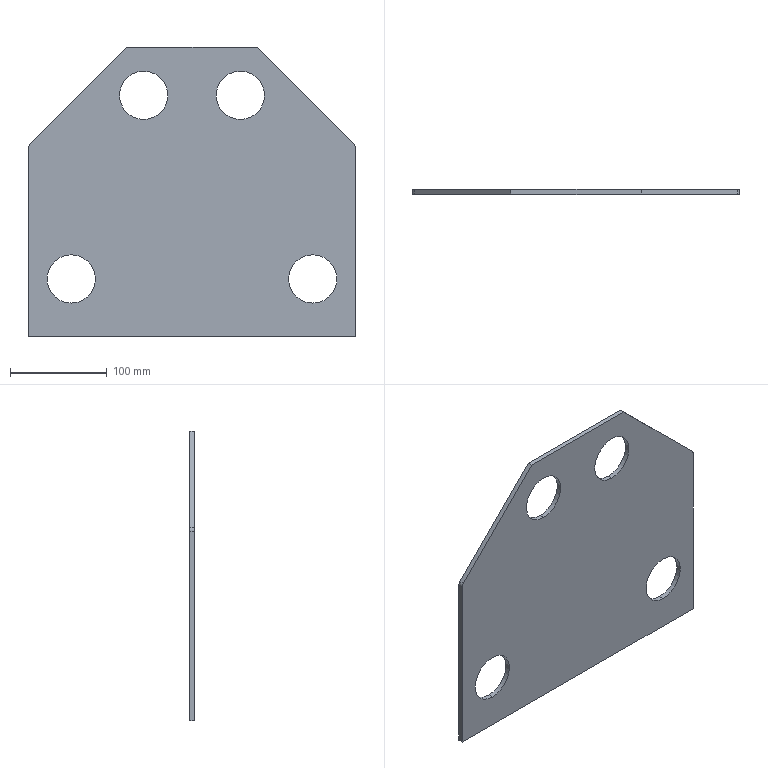Component | SolidWorks | 007PartitionPlate-2 | 1 solid | 18 faces | box 338 x 5 x 300 mm | volume 416213 mm3 | cylinder 10 | plane 8 | commonest cylinder face diameters 50 x8 10 x2 | material Plain Carbon Steel
build123d program:
from build123d import *

# Parameters (mm, degrees)
BOSS_EXTRUDE1_DEPTH = 5
CUT_EXTRUDE1_REACH  = 346.363
SKETCH2_R           = 25
FILLET1_R           = 5


with BuildPart() as part:
    # Sketch1 → Boss-Extrude1 (new body)
    with BuildSketch(Plane.XY):
        Polygon((-198.5, -169), (0, -169), (0, 169), (-198.5, 169), (-300, 67.5), (-300, -67.5), align=None)
    extrude(amount=BOSS_EXTRUDE1_DEPTH)

    # Sketch2 → Cut-Extrude1 (cut, up to next)
    with BuildSketch(Plane.XY.offset(5), mode=Mode.PRIVATE) as cut_extrude1_sk1:
        with Locations((-250, 50)):
            Circle(SKETCH2_R)
    cut_extrude1_tool1 = extrude(cut_extrude1_sk1.sketch, amount=-CUT_EXTRUDE1_REACH, mode=Mode.PRIVATE) & part.part
    # Sketch2 → Cut-Extrude1 (cut, up to next)
    with BuildSketch(Plane.XY.offset(5), mode=Mode.PRIVATE) as cut_extrude1_sk2:
        with Locations((-250, -50)):
            Circle(SKETCH2_R)
    cut_extrude1_tool2 = extrude(cut_extrude1_sk2.sketch, amount=-CUT_EXTRUDE1_REACH, mode=Mode.PRIVATE) & part.part
    # Sketch2 → Cut-Extrude1 (cut, up to next)
    with BuildSketch(Plane.XY.offset(5), mode=Mode.PRIVATE) as cut_extrude1_sk3:
        with Locations((-60, 125)):
            Circle(SKETCH2_R)
    cut_extrude1_tool3 = extrude(cut_extrude1_sk3.sketch, amount=-CUT_EXTRUDE1_REACH, mode=Mode.PRIVATE) & part.part
    # Sketch2 → Cut-Extrude1 (cut, up to next)
    with BuildSketch(Plane.XY.offset(5), mode=Mode.PRIVATE) as cut_extrude1_sk4:
        with Locations((-60, -125)):
            Circle(SKETCH2_R)
    cut_extrude1_tool4 = extrude(cut_extrude1_sk4.sketch, amount=-CUT_EXTRUDE1_REACH, mode=Mode.PRIVATE) & part.part
    add(cut_extrude1_tool1.solids().sort_by_distance((-250, 50, 5))[0], mode=Mode.SUBTRACT)
    add(cut_extrude1_tool2.solids().sort_by_distance((-250, -50, 5))[0], mode=Mode.SUBTRACT)
    add(cut_extrude1_tool3.solids().sort_by_distance((-60, 125, 5))[0], mode=Mode.SUBTRACT)
    add(cut_extrude1_tool4.solids().sort_by_distance((-60, -125, 5))[0], mode=Mode.SUBTRACT)

    # Fillet1
    fillet1_edges = [part.edges().sort_by_distance(p)[0] for p in [
        (-198.5, -169, 2.5),
        (-198.5, 169, 2.5),
    ]]
    fillet(fillet1_edges, radius=FILLET1_R)


solid = part.part

# Placed as in the assembly
solid = solid.moved(Location((130, 1207, -306), (90, 0, -90)))
STEP:
#1=COLOUR_RGB('',0.7922,0.8196,0.9333);
#2=FILL_AREA_STYLE_COLOUR('',#1);
#3=FILL_AREA_STYLE('',(#2));
#4=SURFACE_STYLE_FILL_AREA(#3);
#5=SURFACE_SIDE_STYLE('',(#4));
#6=SURFACE_STYLE_USAGE(.BOTH.,#5);
#7=PRESENTATION_STYLE_ASSIGNMENT((#6));
#8=CARTESIAN_POINT('',(0.1969,47.52,-8.701));
#9=VERTEX_POINT('',#8);
#10=CARTESIAN_POINT('',(0.1969,47.52,-10.669));
#11=VERTEX_POINT('',#10);
#12=CARTESIAN_POINT('',(0.1969,47.52,-9.685));
#13=DIRECTION('',(0.,-1.,0.));
#14=DIRECTION('',(-0.,0.,1.));
#15=AXIS2_PLACEMENT_3D('',#12,#13,#14);
#16=CIRCLE('',#15,0.9843);
#17=EDGE_CURVE('',#9,#11,#16,.T.);
#18=ORIENTED_EDGE('',*,*,#17,.F.);
#19=CARTESIAN_POINT('',(0.1969,47.323,-8.701));
#20=VERTEX_POINT('',#19);
#21=CARTESIAN_POINT('',(0.1969,47.52,-8.701));
#22=DIRECTION('',(0.,-1.,0.));
#23=VECTOR('',#22,39.37);
#24=LINE('',#21,#23);
#25=EDGE_CURVE('',#9,#20,#24,.T.);
#26=ORIENTED_EDGE('',*,*,#25,.T.);
#27=CARTESIAN_POINT('',(0.1969,47.323,-10.669));
#28=VERTEX_POINT('',#27);
#29=CARTESIAN_POINT('',(0.1969,47.323,-9.685));
#30=DIRECTION('',(0.,-1.,0.));
#31=DIRECTION('',(0.,0.,-1.));
#32=AXIS2_PLACEMENT_3D('',#29,#30,#31);
#33=CIRCLE('',#32,0.9843);
#34=EDGE_CURVE('',#20,#28,#33,.T.);
#35=ORIENTED_EDGE('',*,*,#34,.T.);
#36=CARTESIAN_POINT('',(0.1969,47.52,-10.669));
#37=DIRECTION('',(0.,-1.,0.));
#38=VECTOR('',#37,39.37);
#39=LINE('',#36,#38);
#40=EDGE_CURVE('',#11,#28,#39,.T.);
#41=ORIENTED_EDGE('',*,*,#40,.F.);
#42=EDGE_LOOP('',(#18,#26,#35,#41));
#43=FACE_OUTER_BOUND('',#42,.T.);
#44=CARTESIAN_POINT('',(0.1969,47.52,-9.685));
#45=DIRECTION('',(0.,-1.,0.));
#46=DIRECTION('',(0.,0.,-1.));
#47=AXIS2_PLACEMENT_3D('',#44,#45,#46);
#48=CYLINDRICAL_SURFACE('',#47,0.9843);
#49=ADVANCED_FACE('',(#43),#48,.F.);
#50=CARTESIAN_POINT('',(10.039,47.52,-8.701));
#51=VERTEX_POINT('',#50);
#52=CARTESIAN_POINT('',(10.039,47.52,-10.669));
#53=VERTEX_POINT('',#52);
#54=CARTESIAN_POINT('',(10.039,47.52,-9.685));
#55=DIRECTION('',(0.,-1.,0.));
#56=DIRECTION('',(0.,0.,1.));
#57=AXIS2_PLACEMENT_3D('',#54,#55,#56);
#58=CIRCLE('',#57,0.9843);
#59=EDGE_CURVE('',#51,#53,#58,.T.);
#60=ORIENTED_EDGE('',*,*,#59,.F.);
#61=CARTESIAN_POINT('',(10.039,47.323,-8.701));
#62=VERTEX_POINT('',#61);
#63=CARTESIAN_POINT('',(10.039,47.52,-8.701));
#64=DIRECTION('',(0.,-1.,0.));
#65=VECTOR('',#64,39.37);
#66=LINE('',#63,#65);
#67=EDGE_CURVE('',#51,#62,#66,.T.);
#68=ORIENTED_EDGE('',*,*,#67,.T.);
#69=CARTESIAN_POINT('',(10.039,47.323,-10.669));
#70=VERTEX_POINT('',#69);
#71=CARTESIAN_POINT('',(10.039,47.323,-9.685));
#72=DIRECTION('',(0.,-1.,0.));
#73=DIRECTION('',(0.,0.,-1.));
#74=AXIS2_PLACEMENT_3D('',#71,#72,#73);
#75=CIRCLE('',#74,0.9843);
#76=EDGE_CURVE('',#62,#70,#75,.T.);
#77=ORIENTED_EDGE('',*,*,#76,.T.);
#78=CARTESIAN_POINT('',(10.039,47.52,-10.669));
#79=DIRECTION('',(0.,-1.,0.));
#80=VECTOR('',#79,39.37);
#81=LINE('',#78,#80);
#82=EDGE_CURVE('',#53,#70,#81,.T.);
#83=ORIENTED_EDGE('',*,*,#82,.F.);
#84=EDGE_LOOP('',(#60,#68,#77,#83));
#85=FACE_OUTER_BOUND('',#84,.T.);
#86=CARTESIAN_POINT('',(10.039,47.52,-9.685));
#87=DIRECTION('',(0.,-1.,0.));
#88=DIRECTION('',(0.,0.,-1.));
#89=AXIS2_PLACEMENT_3D('',#86,#87,#88);
#90=CYLINDRICAL_SURFACE('',#89,0.9843);
#91=ADVANCED_FACE('',(#85),#90,.F.);
#92=CARTESIAN_POINT('',(3.15,47.52,-1.22));
#93=VERTEX_POINT('',#92);
#94=CARTESIAN_POINT('',(3.15,47.52,-3.189));
#95=VERTEX_POINT('',#94);
#96=CARTESIAN_POINT('',(3.15,47.52,-2.205));
#97=DIRECTION('',(0.,-1.,0.));
#98=DIRECTION('',(0.,0.,1.));
#99=AXIS2_PLACEMENT_3D('',#96,#97,#98);
#100=CIRCLE('',#99,0.9843);
#101=EDGE_CURVE('',#93,#95,#100,.T.);
#102=ORIENTED_EDGE('',*,*,#101,.F.);
#103=CARTESIAN_POINT('',(3.15,47.323,-1.22));
#104=VERTEX_POINT('',#103);
#105=CARTESIAN_POINT('',(3.15,47.52,-1.22));
#106=DIRECTION('',(0.,-1.,0.));
#107=VECTOR('',#106,39.37);
#108=LINE('',#105,#107);
#109=EDGE_CURVE('',#93,#104,#108,.T.);
#110=ORIENTED_EDGE('',*,*,#109,.T.);
#111=CARTESIAN_POINT('',(3.15,47.323,-3.189));
#112=VERTEX_POINT('',#111);
#113=CARTESIAN_POINT('',(3.15,47.323,-2.205));
#114=DIRECTION('',(0.,-1.,0.));
#115=DIRECTION('',(0.,0.,-1.));
#116=AXIS2_PLACEMENT_3D('',#113,#114,#115);
#117=CIRCLE('',#116,0.9843);
#118=EDGE_CURVE('',#104,#112,#117,.T.);
#119=ORIENTED_EDGE('',*,*,#118,.T.);
#120=CARTESIAN_POINT('',(3.15,47.52,-3.189));
#121=DIRECTION('',(0.,-1.,0.));
#122=VECTOR('',#121,39.37);
#123=LINE('',#120,#122);
#124=EDGE_CURVE('',#95,#112,#123,.T.);
#125=ORIENTED_EDGE('',*,*,#124,.F.);
#126=EDGE_LOOP('',(#102,#110,#119,#125));
#127=FACE_OUTER_BOUND('',#126,.T.);
#128=CARTESIAN_POINT('',(3.15,47.52,-2.205));
#129=DIRECTION('',(0.,-1.,0.));
#130=DIRECTION('',(0.,0.,-1.));
#131=AXIS2_PLACEMENT_3D('',#128,#129,#130);
#132=CYLINDRICAL_SURFACE('',#131,0.9843);
#133=ADVANCED_FACE('',(#127),#132,.F.);
#134=CARTESIAN_POINT('',(7.087,47.52,-1.22));
#135=VERTEX_POINT('',#134);
#136=CARTESIAN_POINT('',(7.087,47.52,-3.189));
#137=VERTEX_POINT('',#136);
#138=CARTESIAN_POINT('',(7.087,47.52,-2.205));
#139=DIRECTION('',(0.,-1.,0.));
#140=DIRECTION('',(0.,0.,1.));
#141=AXIS2_PLACEMENT_3D('',#138,#139,#140);
#142=CIRCLE('',#141,0.9843);
#143=EDGE_CURVE('',#135,#137,#142,.T.);
#144=ORIENTED_EDGE('',*,*,#143,.F.);
#145=CARTESIAN_POINT('',(7.087,47.323,-1.22));
#146=VERTEX_POINT('',#145);
#147=CARTESIAN_POINT('',(7.087,47.52,-1.22));
#148=DIRECTION('',(0.,-1.,0.));
#149=VECTOR('',#148,39.37);
#150=LINE('',#147,#149);
#151=EDGE_CURVE('',#135,#146,#150,.T.);
#152=ORIENTED_EDGE('',*,*,#151,.T.);
#153=CARTESIAN_POINT('',(7.087,47.323,-3.189));
#154=VERTEX_POINT('',#153);
#155=CARTESIAN_POINT('',(7.087,47.323,-2.205));
#156=DIRECTION('',(0.,-1.,0.));
#157=DIRECTION('',(0.,0.,-1.));
#158=AXIS2_PLACEMENT_3D('',#155,#156,#157);
#159=CIRCLE('',#158,0.9843);
#160=EDGE_CURVE('',#146,#154,#159,.T.);
#161=ORIENTED_EDGE('',*,*,#160,.T.);
#162=CARTESIAN_POINT('',(7.087,47.52,-3.189));
#163=DIRECTION('',(0.,-1.,0.));
#164=VECTOR('',#163,39.37);
#165=LINE('',#162,#164);
#166=EDGE_CURVE('',#137,#154,#165,.T.);
#167=ORIENTED_EDGE('',*,*,#166,.F.);
#168=EDGE_LOOP('',(#144,#152,#161,#167));
#169=FACE_OUTER_BOUND('',#168,.T.);
#170=CARTESIAN_POINT('',(7.087,47.52,-2.205));
#171=DIRECTION('',(0.,-1.,0.));
#172=DIRECTION('',(0.,0.,-1.));
#173=AXIS2_PLACEMENT_3D('',#170,#171,#172);
#174=CYLINDRICAL_SURFACE('',#173,0.9843);
#175=ADVANCED_FACE('',(#169),#174,.F.);
#176=CARTESIAN_POINT('',(-1.535,47.52,-12.047));
#177=VERTEX_POINT('',#176);
#178=CARTESIAN_POINT('',(11.772,47.52,-12.047));
#179=VERTEX_POINT('',#178);
#180=CARTESIAN_POINT('',(-1.535,47.52,-12.047));
#181=DIRECTION('',(1.,0.,0.));
#182=VECTOR('',#181,39.37);
#183=LINE('',#180,#182);
#184=EDGE_CURVE('',#177,#179,#183,.T.);
#185=ORIENTED_EDGE('',*,*,#184,.T.);
#186=CARTESIAN_POINT('',(11.772,47.323,-12.047));
#187=VERTEX_POINT('',#186);
#188=CARTESIAN_POINT('',(11.772,47.323,-12.047));
#189=DIRECTION('',(0.,1.,0.));
#190=VECTOR('',#189,39.37);
#191=LINE('',#188,#190);
#192=EDGE_CURVE('',#187,#179,#191,.T.);
#193=ORIENTED_EDGE('',*,*,#192,.F.);
#194=CARTESIAN_POINT('',(-1.535,47.323,-12.047));
#195=VERTEX_POINT('',#194);
#196=CARTESIAN_POINT('',(-1.535,47.323,-12.047));
#197=DIRECTION('',(1.,0.,0.));
#198=VECTOR('',#197,39.37);
#199=LINE('',#196,#198);
#200=EDGE_CURVE('',#195,#187,#199,.T.);
#201=ORIENTED_EDGE('',*,*,#200,.F.);
#202=CARTESIAN_POINT('',(-1.535,47.323,-12.047));
#203=DIRECTION('',(0.,1.,0.));
#204=VECTOR('',#203,39.37);
#205=LINE('',#202,#204);
#206=EDGE_CURVE('',#195,#177,#205,.T.);
#207=ORIENTED_EDGE('',*,*,#206,.T.);
#208=EDGE_LOOP('',(#185,#193,#201,#207));
#209=FACE_OUTER_BOUND('',#208,.T.);
#210=CARTESIAN_POINT('',(-1.535,47.323,-12.047));
#211=DIRECTION('',(-0.,0.,1.));
#212=DIRECTION('',(0.,-1.,0.));
#213=AXIS2_PLACEMENT_3D('',#210,#211,#212);
#214=PLANE('',#213);
#215=ADVANCED_FACE('',(#209),#214,.F.);
#216=CARTESIAN_POINT('',(11.772,47.52,-4.314));
#217=VERTEX_POINT('',#216);
#218=CARTESIAN_POINT('',(11.772,47.52,-4.232));
#219=DIRECTION('',(-0.,0.,1.));
#220=VECTOR('',#219,39.37);
#221=LINE('',#218,#220);
#222=EDGE_CURVE('',#179,#217,#221,.T.);
#223=ORIENTED_EDGE('',*,*,#222,.T.);
#224=CARTESIAN_POINT('',(11.772,47.323,-4.314));
#225=VERTEX_POINT('',#224);
#226=CARTESIAN_POINT('',(11.772,47.323,-4.314));
#227=DIRECTION('',(0.,-1.,0.));
#228=VECTOR('',#227,39.37);
#229=LINE('',#226,#228);
#230=EDGE_CURVE('',#217,#225,#229,.T.);
#231=ORIENTED_EDGE('',*,*,#230,.T.);
#232=CARTESIAN_POINT('',(11.772,47.323,-4.232));
#233=DIRECTION('',(-0.,0.,1.));
#234=VECTOR('',#233,39.37);
#235=LINE('',#232,#234);
#236=EDGE_CURVE('',#187,#225,#235,.T.);
#237=ORIENTED_EDGE('',*,*,#236,.F.);
#238=ORIENTED_EDGE('',*,*,#192,.T.);
#239=EDGE_LOOP('',(#223,#231,#237,#238));
#240=FACE_OUTER_BOUND('',#239,.T.);
#241=CARTESIAN_POINT('',(11.772,47.323,-4.232));
#242=DIRECTION('',(-1.,0.,-0.));
#243=DIRECTION('',(0.,1.,0.));
#244=AXIS2_PLACEMENT_3D('',#241,#242,#243);
#245=PLANE('',#244);
#246=ADVANCED_FACE('',(#240),#245,.F.);
#247=CARTESIAN_POINT('',(11.714,47.323,-4.175));
#248=VERTEX_POINT('',#247);
#249=CARTESIAN_POINT('',(7.776,47.323,-0.2362));
#250=VERTEX_POINT('',#249);
#251=CARTESIAN_POINT('',(7.776,47.323,-0.2362));
#252=DIRECTION('',(-0.7071,0.,0.7071));
#253=VECTOR('',#252,39.37);
#254=LINE('',#251,#253);
#255=EDGE_CURVE('',#248,#250,#254,.T.);
#256=ORIENTED_EDGE('',*,*,#255,.F.);
#257=CARTESIAN_POINT('',(11.714,47.52,-4.175));
#258=VERTEX_POINT('',#257);
#259=CARTESIAN_POINT('',(11.714,47.323,-4.175));
#260=DIRECTION('',(0.,1.,0.));
#261=VECTOR('',#260,39.37);
#262=LINE('',#259,#261);
#263=EDGE_CURVE('',#248,#258,#262,.T.);
#264=ORIENTED_EDGE('',*,*,#263,.T.);
#265=CARTESIAN_POINT('',(7.776,47.52,-0.2362));
#266=VERTEX_POINT('',#265);
#267=CARTESIAN_POINT('',(7.776,47.52,-0.2362));
#268=DIRECTION('',(-0.7071,0.,0.7071));
#269=VECTOR('',#268,39.37);
#270=LINE('',#267,#269);
#271=EDGE_CURVE('',#258,#266,#270,.T.);
#272=ORIENTED_EDGE('',*,*,#271,.T.);
#273=CARTESIAN_POINT('',(7.776,47.323,-0.2362));
#274=DIRECTION('',(0.,1.,0.));
#275=VECTOR('',#274,39.37);
#276=LINE('',#273,#275);
#277=EDGE_CURVE('',#250,#266,#276,.T.);
#278=ORIENTED_EDGE('',*,*,#277,.F.);
#279=EDGE_LOOP('',(#256,#264,#272,#278));
#280=FACE_OUTER_BOUND('',#279,.T.);
#281=CARTESIAN_POINT('',(7.776,47.323,-0.2362));
#282=DIRECTION('',(-0.7071,0.,-0.7071));
#283=DIRECTION('',(0.7071,0.,-0.7071));
#284=AXIS2_PLACEMENT_3D('',#281,#282,#283);
#285=PLANE('',#284);
#286=ADVANCED_FACE('',(#280),#285,.F.);
#287=CARTESIAN_POINT('',(2.461,47.52,-0.2362));
#288=VERTEX_POINT('',#287);
#289=CARTESIAN_POINT('',(2.461,47.52,-0.2362));
#290=DIRECTION('',(-1.,0.,-0.));
#291=VECTOR('',#290,39.37);
#292=LINE('',#289,#291);
#293=EDGE_CURVE('',#266,#288,#292,.T.);
#294=ORIENTED_EDGE('',*,*,#293,.T.);
#295=CARTESIAN_POINT('',(2.461,47.323,-0.2362));
#296=VERTEX_POINT('',#295);
#297=CARTESIAN_POINT('',(2.461,47.323,-0.2362));
#298=DIRECTION('',(0.,1.,0.));
#299=VECTOR('',#298,39.37);
#300=LINE('',#297,#299);
#301=EDGE_CURVE('',#296,#288,#300,.T.);
#302=ORIENTED_EDGE('',*,*,#301,.F.);
#303=CARTESIAN_POINT('',(2.461,47.323,-0.2362));
#304=DIRECTION('',(-1.,0.,-0.));
#305=VECTOR('',#304,39.37);
#306=LINE('',#303,#305);
#307=EDGE_CURVE('',#250,#296,#306,.T.);
#308=ORIENTED_EDGE('',*,*,#307,.F.);
#309=ORIENTED_EDGE('',*,*,#277,.T.);
#310=EDGE_LOOP('',(#294,#302,#308,#309));
#311=FACE_OUTER_BOUND('',#310,.T.);
#312=CARTESIAN_POINT('',(2.461,47.323,-0.2362));
#313=DIRECTION('',(0.,0.,-1.));
#314=DIRECTION('',(0.,1.,0.));
#315=AXIS2_PLACEMENT_3D('',#312,#313,#314);
#316=PLANE('',#315);
#317=ADVANCED_FACE('',(#311),#316,.F.);
#318=CARTESIAN_POINT('',(-1.478,47.52,-4.175));
#319=VERTEX_POINT('',#318);
#320=CARTESIAN_POINT('',(2.461,47.52,-0.2362));
#321=DIRECTION('',(-0.7071,0.,-0.7071));
#322=VECTOR('',#321,39.37);
#323=LINE('',#320,#322);
#324=EDGE_CURVE('',#288,#319,#323,.T.);
#325=ORIENTED_EDGE('',*,*,#324,.T.);
#326=CARTESIAN_POINT('',(-1.478,47.323,-4.175));
#327=VERTEX_POINT('',#326);
#328=CARTESIAN_POINT('',(-1.478,47.323,-4.175));
#329=DIRECTION('',(0.,-1.,0.));
#330=VECTOR('',#329,39.37);
#331=LINE('',#328,#330);
#332=EDGE_CURVE('',#319,#327,#331,.T.);
#333=ORIENTED_EDGE('',*,*,#332,.T.);
#334=CARTESIAN_POINT('',(2.461,47.323,-0.2362));
#335=DIRECTION('',(-0.7071,0.,-0.7071));
#336=VECTOR('',#335,39.37);
#337=LINE('',#334,#336);
#338=EDGE_CURVE('',#296,#327,#337,.T.);
#339=ORIENTED_EDGE('',*,*,#338,.F.);
#340=ORIENTED_EDGE('',*,*,#301,.T.);
#341=EDGE_LOOP('',(#325,#333,#339,#340));
#342=FACE_OUTER_BOUND('',#341,.T.);
#343=CARTESIAN_POINT('',(2.461,47.323,-0.2362));
#344=DIRECTION('',(0.7071,0.,-0.7071));
#345=DIRECTION('',(0.7071,0.,0.7071));
#346=AXIS2_PLACEMENT_3D('',#343,#344,#345);
#347=PLANE('',#346);
#348=ADVANCED_FACE('',(#342),#347,.F.);
#349=CARTESIAN_POINT('',(-1.535,47.323,-4.314));
#350=VERTEX_POINT('',#349);
#351=CARTESIAN_POINT('',(-1.535,47.323,-4.232));
#352=DIRECTION('',(0.,0.,-1.));
#353=VECTOR('',#352,39.37);
#354=LINE('',#351,#353);
#355=EDGE_CURVE('',#350,#195,#354,.T.);
#356=ORIENTED_EDGE('',*,*,#355,.F.);
#357=CARTESIAN_POINT('',(-1.535,47.52,-4.314));
#358=VERTEX_POINT('',#357);
#359=CARTESIAN_POINT('',(-1.535,47.323,-4.314));
#360=DIRECTION('',(0.,1.,0.));
#361=VECTOR('',#360,39.37);
#362=LINE('',#359,#361);
#363=EDGE_CURVE('',#350,#358,#362,.T.);
#364=ORIENTED_EDGE('',*,*,#363,.T.);
#365=CARTESIAN_POINT('',(-1.535,47.52,-4.232));
#366=DIRECTION('',(0.,0.,-1.));
#367=VECTOR('',#366,39.37);
#368=LINE('',#365,#367);
#369=EDGE_CURVE('',#358,#177,#368,.T.);
#370=ORIENTED_EDGE('',*,*,#369,.T.);
#371=ORIENTED_EDGE('',*,*,#206,.F.);
#372=EDGE_LOOP('',(#356,#364,#370,#371));
#373=FACE_OUTER_BOUND('',#372,.T.);
#374=CARTESIAN_POINT('',(-1.535,47.323,-4.232));
#375=DIRECTION('',(1.,0.,0.));
#376=DIRECTION('',(0.,-1.,0.));
#377=AXIS2_PLACEMENT_3D('',#374,#375,#376);
#378=PLANE('',#377);
#379=ADVANCED_FACE('',(#373),#378,.F.);
#380=CARTESIAN_POINT('',(0.1969,47.323,-9.685));
#381=DIRECTION('',(0.,-1.,0.));
#382=DIRECTION('',(0.,0.,-1.));
#383=AXIS2_PLACEMENT_3D('',#380,#381,#382);
#384=CIRCLE('',#383,0.9843);
#385=EDGE_CURVE('',#28,#20,#384,.T.);
#386=ORIENTED_EDGE('',*,*,#385,.F.);
#387=ORIENTED_EDGE('',*,*,#34,.F.);
#388=EDGE_LOOP('',(#386,#387));
#389=FACE_BOUND('',#388,.T.);
#390=CARTESIAN_POINT('',(10.039,47.323,-9.685));
#391=DIRECTION('',(0.,-1.,0.));
#392=DIRECTION('',(0.,0.,-1.));
#393=AXIS2_PLACEMENT_3D('',#390,#391,#392);
#394=CIRCLE('',#393,0.9843);
#395=EDGE_CURVE('',#70,#62,#394,.T.);
#396=ORIENTED_EDGE('',*,*,#395,.F.);
#397=ORIENTED_EDGE('',*,*,#76,.F.);
#398=EDGE_LOOP('',(#396,#397));
#399=FACE_BOUND('',#398,.T.);
#400=CARTESIAN_POINT('',(3.15,47.323,-2.205));
#401=DIRECTION('',(0.,-1.,0.));
#402=DIRECTION('',(0.,0.,-1.));
#403=AXIS2_PLACEMENT_3D('',#400,#401,#402);
#404=CIRCLE('',#403,0.9843);
#405=EDGE_CURVE('',#112,#104,#404,.T.);
#406=ORIENTED_EDGE('',*,*,#405,.F.);
#407=ORIENTED_EDGE('',*,*,#118,.F.);
#408=EDGE_LOOP('',(#406,#407));
#409=FACE_BOUND('',#408,.T.);
#410=CARTESIAN_POINT('',(7.087,47.323,-2.205));
#411=DIRECTION('',(0.,-1.,0.));
#412=DIRECTION('',(0.,0.,-1.));
#413=AXIS2_PLACEMENT_3D('',#410,#411,#412);
#414=CIRCLE('',#413,0.9843);
#415=EDGE_CURVE('',#154,#146,#414,.T.);
#416=ORIENTED_EDGE('',*,*,#415,.F.);
#417=ORIENTED_EDGE('',*,*,#160,.F.);
#418=EDGE_LOOP('',(#416,#417));
#419=FACE_BOUND('',#418,.T.);
#420=ORIENTED_EDGE('',*,*,#338,.T.);
#421=CARTESIAN_POINT('',(-1.339,47.323,-4.314));
#422=DIRECTION('',(0.,-1.,0.));
#423=DIRECTION('',(0.,0.,1.));
#424=AXIS2_PLACEMENT_3D('',#421,#422,#423);
#425=CIRCLE('',#424,0.1969);
#426=EDGE_CURVE('',#327,#350,#425,.T.);
#427=ORIENTED_EDGE('',*,*,#426,.T.);
#428=ORIENTED_EDGE('',*,*,#355,.T.);
#429=ORIENTED_EDGE('',*,*,#200,.T.);
#430=ORIENTED_EDGE('',*,*,#236,.T.);
#431=CARTESIAN_POINT('',(11.575,47.323,-4.314));
#432=DIRECTION('',(0.,-1.,0.));
#433=DIRECTION('',(0.,0.,1.));
#434=AXIS2_PLACEMENT_3D('',#431,#432,#433);
#435=CIRCLE('',#434,0.1969);
#436=EDGE_CURVE('',#225,#248,#435,.T.);
#437=ORIENTED_EDGE('',*,*,#436,.T.);
#438=ORIENTED_EDGE('',*,*,#255,.T.);
#439=ORIENTED_EDGE('',*,*,#307,.T.);
#440=EDGE_LOOP('',(#420,#427,#428,#429,#430,#437,#438,#439));
#441=FACE_OUTER_BOUND('',#440,.T.);
#442=CARTESIAN_POINT('',(11.772,47.323,-12.047));
#443=DIRECTION('',(0.,1.,0.));
#444=DIRECTION('',(-0.,0.,1.));
#445=AXIS2_PLACEMENT_3D('',#442,#443,#444);
#446=PLANE('',#445);
#447=ADVANCED_FACE('',(#389,#399,#409,#419,#441),#446,.F.);
#448=CARTESIAN_POINT('',(0.1969,47.52,-9.685));
#449=DIRECTION('',(0.,-1.,0.));
#450=DIRECTION('',(-0.,0.,1.));
#451=AXIS2_PLACEMENT_3D('',#448,#449,#450);
#452=CIRCLE('',#451,0.9843);
#453=EDGE_CURVE('',#11,#9,#452,.T.);
#454=ORIENTED_EDGE('',*,*,#453,.T.);
#455=ORIENTED_EDGE('',*,*,#17,.T.);
#456=EDGE_LOOP('',(#454,#455));
#457=FACE_BOUND('',#456,.T.);
#458=CARTESIAN_POINT('',(10.039,47.52,-9.685));
#459=DIRECTION('',(0.,-1.,0.));
#460=DIRECTION('',(0.,0.,1.));
#461=AXIS2_PLACEMENT_3D('',#458,#459,#460);
#462=CIRCLE('',#461,0.9843);
#463=EDGE_CURVE('',#53,#51,#462,.T.);
#464=ORIENTED_EDGE('',*,*,#463,.T.);
#465=ORIENTED_EDGE('',*,*,#59,.T.);
#466=EDGE_LOOP('',(#464,#465));
#467=FACE_BOUND('',#466,.T.);
#468=CARTESIAN_POINT('',(3.15,47.52,-2.205));
#469=DIRECTION('',(0.,-1.,0.));
#470=DIRECTION('',(0.,0.,1.));
#471=AXIS2_PLACEMENT_3D('',#468,#469,#470);
#472=CIRCLE('',#471,0.9843);
#473=EDGE_CURVE('',#95,#93,#472,.T.);
#474=ORIENTED_EDGE('',*,*,#473,.T.);
#475=ORIENTED_EDGE('',*,*,#101,.T.);
#476=EDGE_LOOP('',(#474,#475));
#477=FACE_BOUND('',#476,.T.);
#478=CARTESIAN_POINT('',(7.087,47.52,-2.205));
#479=DIRECTION('',(0.,-1.,0.));
#480=DIRECTION('',(0.,0.,1.));
#481=AXIS2_PLACEMENT_3D('',#478,#479,#480);
#482=CIRCLE('',#481,0.9843);
#483=EDGE_CURVE('',#137,#135,#482,.T.);
#484=ORIENTED_EDGE('',*,*,#483,.T.);
#485=ORIENTED_EDGE('',*,*,#143,.T.);
#486=EDGE_LOOP('',(#484,#485));
#487=FACE_BOUND('',#486,.T.);
#488=ORIENTED_EDGE('',*,*,#369,.F.);
#489=CARTESIAN_POINT('',(-1.339,47.52,-4.314));
#490=DIRECTION('',(0.,1.,0.));
#491=DIRECTION('',(0.,0.,1.));
#492=AXIS2_PLACEMENT_3D('',#489,#490,#491);
#493=CIRCLE('',#492,0.1969);
#494=EDGE_CURVE('',#358,#319,#493,.T.);
#495=ORIENTED_EDGE('',*,*,#494,.T.);
#496=ORIENTED_EDGE('',*,*,#324,.F.);
#497=ORIENTED_EDGE('',*,*,#293,.F.);
#498=ORIENTED_EDGE('',*,*,#271,.F.);
#499=CARTESIAN_POINT('',(11.575,47.52,-4.314));
#500=DIRECTION('',(0.,1.,0.));
#501=DIRECTION('',(0.,0.,1.));
#502=AXIS2_PLACEMENT_3D('',#499,#500,#501);
#503=CIRCLE('',#502,0.1969);
#504=EDGE_CURVE('',#258,#217,#503,.T.);
#505=ORIENTED_EDGE('',*,*,#504,.T.);
#506=ORIENTED_EDGE('',*,*,#222,.F.);
#507=ORIENTED_EDGE('',*,*,#184,.F.);
#508=EDGE_LOOP('',(#488,#495,#496,#497,#498,#505,#506,#507));
#509=FACE_OUTER_BOUND('',#508,.T.);
#510=CARTESIAN_POINT('',(11.772,47.52,-12.047));
#511=DIRECTION('',(0.,1.,0.));
#512=DIRECTION('',(-0.,0.,1.));
#513=AXIS2_PLACEMENT_3D('',#510,#511,#512);
#514=PLANE('',#513);
#515=ADVANCED_FACE('',(#457,#467,#477,#487,#509),#514,.T.);
#516=ORIENTED_EDGE('',*,*,#151,.F.);
#517=ORIENTED_EDGE('',*,*,#483,.F.);
#518=ORIENTED_EDGE('',*,*,#166,.T.);
#519=ORIENTED_EDGE('',*,*,#415,.T.);
#520=EDGE_LOOP('',(#516,#517,#518,#519));
#521=FACE_OUTER_BOUND('',#520,.T.);
#522=CARTESIAN_POINT('',(7.087,47.52,-2.205));
#523=DIRECTION('',(0.,-1.,0.));
#524=DIRECTION('',(0.,0.,-1.));
#525=AXIS2_PLACEMENT_3D('',#522,#523,#524);
#526=CYLINDRICAL_SURFACE('',#525,0.9843);
#527=ADVANCED_FACE('',(#521),#526,.F.);
#528=ORIENTED_EDGE('',*,*,#109,.F.);
#529=ORIENTED_EDGE('',*,*,#473,.F.);
#530=ORIENTED_EDGE('',*,*,#124,.T.);
#531=ORIENTED_EDGE('',*,*,#405,.T.);
#532=EDGE_LOOP('',(#528,#529,#530,#531));
#533=FACE_OUTER_BOUND('',#532,.T.);
#534=CARTESIAN_POINT('',(3.15,47.52,-2.205));
#535=DIRECTION('',(0.,-1.,0.));
#536=DIRECTION('',(0.,0.,-1.));
#537=AXIS2_PLACEMENT_3D('',#534,#535,#536);
#538=CYLINDRICAL_SURFACE('',#537,0.9843);
#539=ADVANCED_FACE('',(#533),#538,.F.);
#540=ORIENTED_EDGE('',*,*,#67,.F.);
#541=ORIENTED_EDGE('',*,*,#463,.F.);
#542=ORIENTED_EDGE('',*,*,#82,.T.);
#543=ORIENTED_EDGE('',*,*,#395,.T.);
#544=EDGE_LOOP('',(#540,#541,#542,#543));
#545=FACE_OUTER_BOUND('',#544,.T.);
#546=CARTESIAN_POINT('',(10.039,47.52,-9.685));
#547=DIRECTION('',(0.,-1.,0.));
#548=DIRECTION('',(0.,0.,-1.));
#549=AXIS2_PLACEMENT_3D('',#546,#547,#548);
#550=CYLINDRICAL_SURFACE('',#549,0.9843);
#551=ADVANCED_FACE('',(#545),#550,.F.);
#552=ORIENTED_EDGE('',*,*,#25,.F.);
#553=ORIENTED_EDGE('',*,*,#453,.F.);
#554=ORIENTED_EDGE('',*,*,#40,.T.);
#555=ORIENTED_EDGE('',*,*,#385,.T.);
#556=EDGE_LOOP('',(#552,#553,#554,#555));
#557=FACE_OUTER_BOUND('',#556,.T.);
#558=CARTESIAN_POINT('',(0.1969,47.52,-9.685));
#559=DIRECTION('',(0.,-1.,0.));
#560=DIRECTION('',(0.,0.,-1.));
#561=AXIS2_PLACEMENT_3D('',#558,#559,#560);
#562=CYLINDRICAL_SURFACE('',#561,0.9843);
#563=ADVANCED_FACE('',(#557),#562,.F.);
#564=ORIENTED_EDGE('',*,*,#426,.F.);
#565=ORIENTED_EDGE('',*,*,#332,.F.);
#566=ORIENTED_EDGE('',*,*,#494,.F.);
#567=ORIENTED_EDGE('',*,*,#363,.F.);
#568=EDGE_LOOP('',(#564,#565,#566,#567));
#569=FACE_OUTER_BOUND('',#568,.T.);
#570=CARTESIAN_POINT('',(-1.339,47.323,-4.314));
#571=DIRECTION('',(0.,1.,0.));
#572=DIRECTION('',(0.,0.,1.));
#573=AXIS2_PLACEMENT_3D('',#570,#571,#572);
#574=CYLINDRICAL_SURFACE('',#573,0.1969);
#575=ADVANCED_FACE('',(#569),#574,.T.);
#576=ORIENTED_EDGE('',*,*,#436,.F.);
#577=ORIENTED_EDGE('',*,*,#230,.F.);
#578=ORIENTED_EDGE('',*,*,#504,.F.);
#579=ORIENTED_EDGE('',*,*,#263,.F.);
#580=EDGE_LOOP('',(#576,#577,#578,#579));
#581=FACE_OUTER_BOUND('',#580,.T.);
#582=CARTESIAN_POINT('',(11.575,47.323,-4.314));
#583=DIRECTION('',(0.,1.,0.));
#584=DIRECTION('',(0.,0.,1.));
#585=AXIS2_PLACEMENT_3D('',#582,#583,#584);
#586=CYLINDRICAL_SURFACE('',#585,0.1969);
#587=ADVANCED_FACE('',(#581),#586,.T.);
#588=CLOSED_SHELL('',(#49,#91,#133,#175,#215,#246,#286,#317,#348,#379,#447,#515,#527,#539,#551,#563,#575,#587));
#589=MANIFOLD_SOLID_BREP('',#588);
#590=STYLED_ITEM('',(#7),#589);
#591=PRESENTATION_LAYER_ASSIGNMENT('','',(#590));
#592=(LENGTH_UNIT()NAMED_UNIT(*)SI_UNIT($,.METRE.));
#593=LENGTH_MEASURE_WITH_UNIT(LENGTH_MEASURE(0.0254),#592);
#594=DIMENSIONAL_EXPONENTS(1.,0.,0.,0.,0.,0.,0.);
#595=(CONVERSION_BASED_UNIT('',#593)LENGTH_UNIT()NAMED_UNIT(#594));
#596=UNCERTAINTY_MEASURE_WITH_UNIT(LENGTH_MEASURE(0.00001),#595,'','');
#597=(NAMED_UNIT(*)PLANE_ANGLE_UNIT()SI_UNIT($,.RADIAN.));
#598=(NAMED_UNIT(*)SI_UNIT($,.STERADIAN.)SOLID_ANGLE_UNIT());
#599=(GEOMETRIC_REPRESENTATION_CONTEXT(3)GLOBAL_UNCERTAINTY_ASSIGNED_CONTEXT((#596))GLOBAL_UNIT_ASSIGNED_CONTEXT((#595,#597,#598))REPRESENTATION_CONTEXT('',''));
#600=MECHANICAL_DESIGN_GEOMETRIC_PRESENTATION_REPRESENTATION('',(#590),#599);
#601=CARTESIAN_POINT('',(0.,0.,0.));
#602=DIRECTION('',(0.,0.,1.));
#603=DIRECTION('',(1.,0.,0.));
#604=AXIS2_PLACEMENT_3D('',#601,#602,#603);
#605=(LENGTH_UNIT()NAMED_UNIT(*)SI_UNIT($,.METRE.));
#606=LENGTH_MEASURE_WITH_UNIT(LENGTH_MEASURE(0.0254),#605);
#607=DIMENSIONAL_EXPONENTS(1.,0.,0.,0.,0.,0.,0.);
#608=(CONVERSION_BASED_UNIT('',#606)LENGTH_UNIT()NAMED_UNIT(#607));
#609=UNCERTAINTY_MEASURE_WITH_UNIT(LENGTH_MEASURE(0.00001),#608,'','');
#610=(NAMED_UNIT(*)PLANE_ANGLE_UNIT()SI_UNIT($,.RADIAN.));
#611=(NAMED_UNIT(*)SI_UNIT($,.STERADIAN.)SOLID_ANGLE_UNIT());
#612=(GEOMETRIC_REPRESENTATION_CONTEXT(3)GLOBAL_UNCERTAINTY_ASSIGNED_CONTEXT((#609))GLOBAL_UNIT_ASSIGNED_CONTEXT((#608,#610,#611))REPRESENTATION_CONTEXT('',''));
#613=ADVANCED_BREP_SHAPE_REPRESENTATION('',(#589,#604),#612);